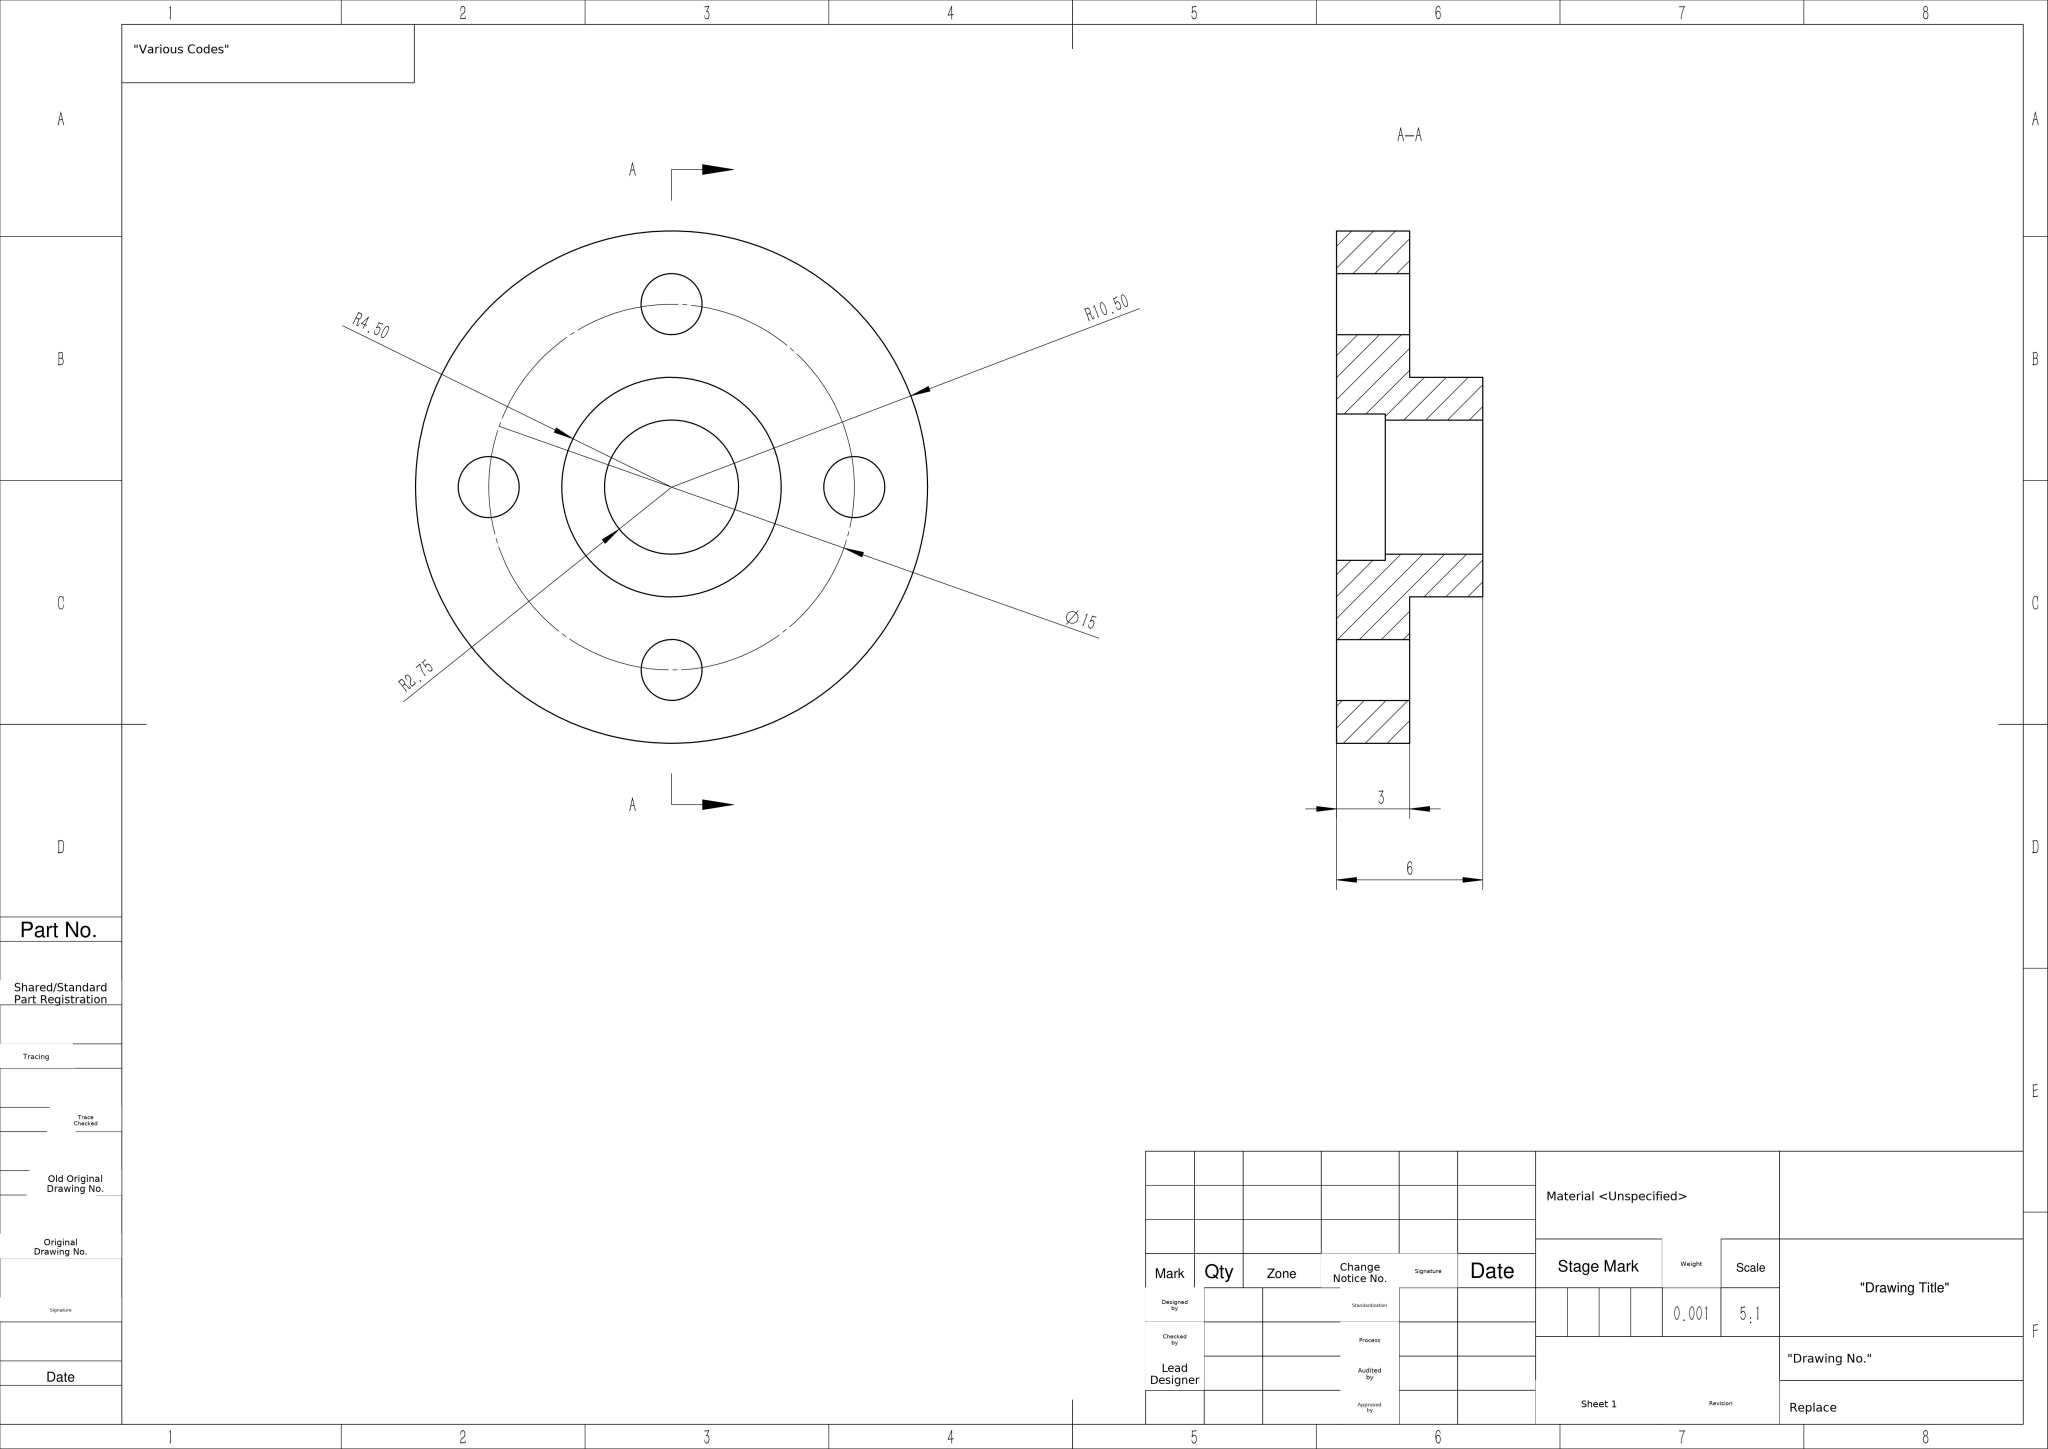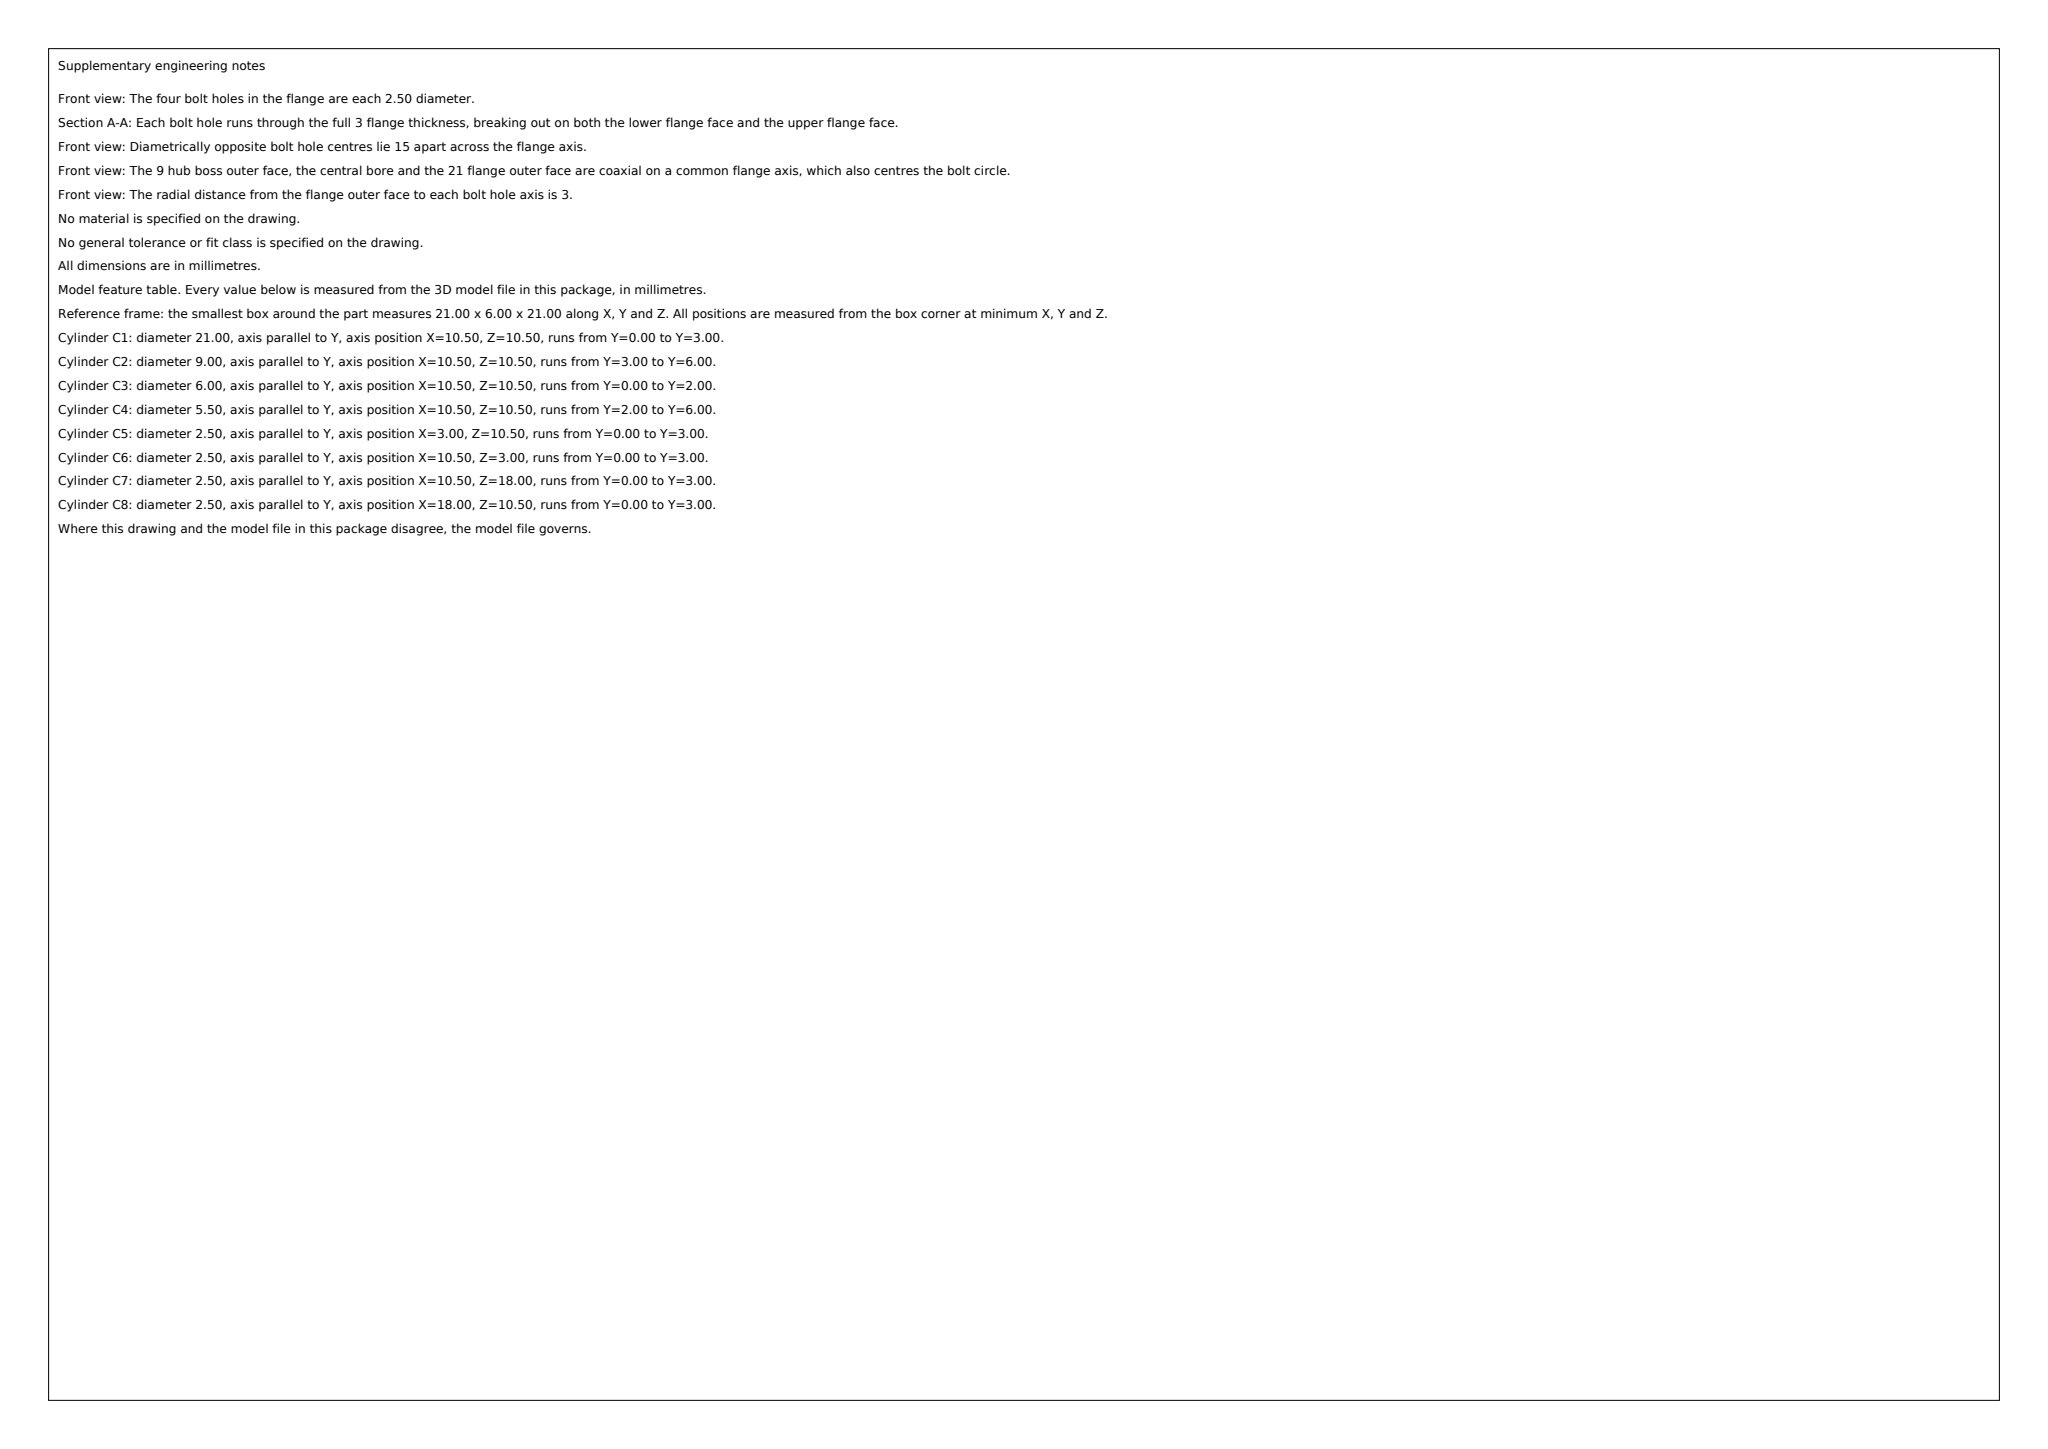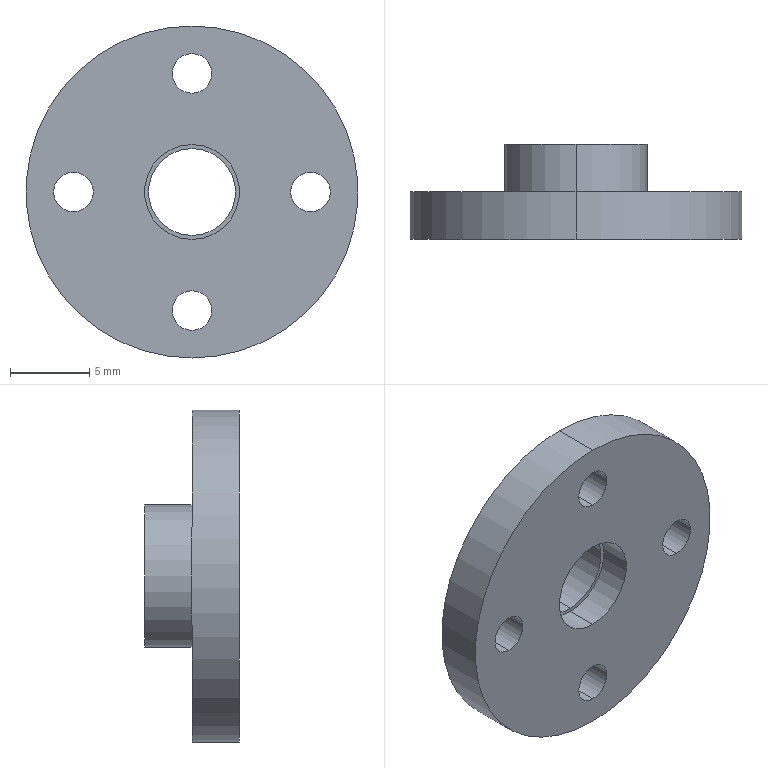Part | SolidWorks | mm | 1 solid | 20 faces | box 21 x 6 x 21 mm | volume 1019 mm3 | cylinder 16 | plane 4 | commonest cylinder face diameters 2.5 x8 6 x2 5.5 x2 9 x2 21 x2
Drawing notes:
Ø5.50 THRU; Ø6.00 DP 2 FROM FLANGE BACK FACE | from the solid: hole/bore dia 5.5 axis y from 2.0 to 6.0 at [10.5,10.5]; hole/bore dia 6.0 axis y from 0.0 to 2.0 at [10.5,10.5]
Ø5.50 THRU FROM Ø6.00 C'BORE FLOOR | from the solid: hole/bore dia 5.5, axis y at (10.5,10.5), from y=2.0 to 6.0 (thru hub end face at y=6); adjacent hole/bore dia 6.0 from y=0 to 2.0
STEP:
#1=CARTESIAN_POINT('',(-0.,3.,-6.25));
#2=VERTEX_POINT('',#1);
#3=CARTESIAN_POINT('',(-0.,0.,-6.25));
#4=VERTEX_POINT('',#3);
#5=CARTESIAN_POINT('',(-0.,6.,-6.25));
#6=DIRECTION('',(0.,-1.,0.));
#7=VECTOR('',#6,1000.);
#8=LINE('',#5,#7);
#9=EDGE_CURVE('',#2,#4,#8,.T.);
#10=ORIENTED_EDGE('',*,*,#9,.F.);
#11=CARTESIAN_POINT('',(-0.,3.,-8.75));
#12=VERTEX_POINT('',#11);
#13=CARTESIAN_POINT('',(-0.,3.,-7.5));
#14=DIRECTION('',(0.,1.,0.));
#15=DIRECTION('',(0.,0.,1.));
#16=AXIS2_PLACEMENT_3D('',#13,#14,#15);
#17=CIRCLE('',#16,1.25);
#18=EDGE_CURVE('',#2,#12,#17,.T.);
#19=ORIENTED_EDGE('',*,*,#18,.T.);
#20=CARTESIAN_POINT('',(-0.,0.,-8.75));
#21=VERTEX_POINT('',#20);
#22=CARTESIAN_POINT('',(-0.,6.,-8.75));
#23=DIRECTION('',(0.,-1.,0.));
#24=VECTOR('',#23,1000.);
#25=LINE('',#22,#24);
#26=EDGE_CURVE('',#12,#21,#25,.T.);
#27=ORIENTED_EDGE('',*,*,#26,.T.);
#28=CARTESIAN_POINT('',(-0.,0.,-7.5));
#29=DIRECTION('',(0.,-1.,0.));
#30=DIRECTION('',(-1.,0.,0.));
#31=AXIS2_PLACEMENT_3D('',#28,#29,#30);
#32=CIRCLE('',#31,1.25);
#33=EDGE_CURVE('',#21,#4,#32,.T.);
#34=ORIENTED_EDGE('',*,*,#33,.T.);
#35=EDGE_LOOP('',(#10,#19,#27,#34));
#36=FACE_OUTER_BOUND('',#35,.T.);
#37=CARTESIAN_POINT('',(-0.,6.,-7.5));
#38=DIRECTION('',(0.,-1.,0.));
#39=DIRECTION('',(0.,0.,-1.));
#40=AXIS2_PLACEMENT_3D('',#37,#38,#39);
#41=CYLINDRICAL_SURFACE('',#40,1.25);
#42=ADVANCED_FACE('',(#36),#41,.F.);
#43=CARTESIAN_POINT('',(-7.5,3.,1.25));
#44=VERTEX_POINT('',#43);
#45=CARTESIAN_POINT('',(-7.5,0.,1.25));
#46=VERTEX_POINT('',#45);
#47=CARTESIAN_POINT('',(-7.5,6.,1.25));
#48=DIRECTION('',(0.,-1.,0.));
#49=VECTOR('',#48,1000.);
#50=LINE('',#47,#49);
#51=EDGE_CURVE('',#44,#46,#50,.T.);
#52=ORIENTED_EDGE('',*,*,#51,.F.);
#53=CARTESIAN_POINT('',(-7.5,3.,-1.25));
#54=VERTEX_POINT('',#53);
#55=CARTESIAN_POINT('',(-7.5,3.,0.));
#56=DIRECTION('',(0.,1.,0.));
#57=DIRECTION('',(0.,0.,1.));
#58=AXIS2_PLACEMENT_3D('',#55,#56,#57);
#59=CIRCLE('',#58,1.25);
#60=EDGE_CURVE('',#44,#54,#59,.T.);
#61=ORIENTED_EDGE('',*,*,#60,.T.);
#62=CARTESIAN_POINT('',(-7.5,0.,-1.25));
#63=VERTEX_POINT('',#62);
#64=CARTESIAN_POINT('',(-7.5,6.,-1.25));
#65=DIRECTION('',(0.,-1.,0.));
#66=VECTOR('',#65,1000.);
#67=LINE('',#64,#66);
#68=EDGE_CURVE('',#54,#63,#67,.T.);
#69=ORIENTED_EDGE('',*,*,#68,.T.);
#70=CARTESIAN_POINT('',(-7.5,0.,0.));
#71=DIRECTION('',(0.,-1.,0.));
#72=DIRECTION('',(0.,0.,1.));
#73=AXIS2_PLACEMENT_3D('',#70,#71,#72);
#74=CIRCLE('',#73,1.25);
#75=EDGE_CURVE('',#63,#46,#74,.T.);
#76=ORIENTED_EDGE('',*,*,#75,.T.);
#77=EDGE_LOOP('',(#52,#61,#69,#76));
#78=FACE_OUTER_BOUND('',#77,.T.);
#79=CARTESIAN_POINT('',(-7.5,6.,0.));
#80=DIRECTION('',(0.,-1.,0.));
#81=DIRECTION('',(0.,0.,-1.));
#82=AXIS2_PLACEMENT_3D('',#79,#80,#81);
#83=CYLINDRICAL_SURFACE('',#82,1.25);
#84=ADVANCED_FACE('',(#78),#83,.F.);
#85=CARTESIAN_POINT('',(0.,3.,8.75));
#86=VERTEX_POINT('',#85);
#87=CARTESIAN_POINT('',(0.,0.,8.75));
#88=VERTEX_POINT('',#87);
#89=CARTESIAN_POINT('',(0.,6.,8.75));
#90=DIRECTION('',(0.,-1.,0.));
#91=VECTOR('',#90,1000.);
#92=LINE('',#89,#91);
#93=EDGE_CURVE('',#86,#88,#92,.T.);
#94=ORIENTED_EDGE('',*,*,#93,.F.);
#95=CARTESIAN_POINT('',(0.,3.,6.25));
#96=VERTEX_POINT('',#95);
#97=CARTESIAN_POINT('',(0.,3.,7.5));
#98=DIRECTION('',(0.,1.,0.));
#99=DIRECTION('',(0.,0.,1.));
#100=AXIS2_PLACEMENT_3D('',#97,#98,#99);
#101=CIRCLE('',#100,1.25);
#102=EDGE_CURVE('',#86,#96,#101,.T.);
#103=ORIENTED_EDGE('',*,*,#102,.T.);
#104=CARTESIAN_POINT('',(0.,0.,6.25));
#105=VERTEX_POINT('',#104);
#106=CARTESIAN_POINT('',(0.,6.,6.25));
#107=DIRECTION('',(0.,-1.,0.));
#108=VECTOR('',#107,1000.);
#109=LINE('',#106,#108);
#110=EDGE_CURVE('',#96,#105,#109,.T.);
#111=ORIENTED_EDGE('',*,*,#110,.T.);
#112=CARTESIAN_POINT('',(0.,0.,7.5));
#113=DIRECTION('',(0.,-1.,0.));
#114=DIRECTION('',(1.,0.,-0.));
#115=AXIS2_PLACEMENT_3D('',#112,#113,#114);
#116=CIRCLE('',#115,1.25);
#117=EDGE_CURVE('',#105,#88,#116,.T.);
#118=ORIENTED_EDGE('',*,*,#117,.T.);
#119=EDGE_LOOP('',(#94,#103,#111,#118));
#120=FACE_OUTER_BOUND('',#119,.T.);
#121=CARTESIAN_POINT('',(0.,6.,7.5));
#122=DIRECTION('',(0.,-1.,0.));
#123=DIRECTION('',(0.,0.,-1.));
#124=AXIS2_PLACEMENT_3D('',#121,#122,#123);
#125=CYLINDRICAL_SURFACE('',#124,1.25);
#126=ADVANCED_FACE('',(#120),#125,.F.);
#127=CARTESIAN_POINT('',(7.5,3.,1.25));
#128=VERTEX_POINT('',#127);
#129=CARTESIAN_POINT('',(7.5,0.,1.25));
#130=VERTEX_POINT('',#129);
#131=CARTESIAN_POINT('',(7.5,6.,1.25));
#132=DIRECTION('',(0.,-1.,0.));
#133=VECTOR('',#132,1000.);
#134=LINE('',#131,#133);
#135=EDGE_CURVE('',#128,#130,#134,.T.);
#136=ORIENTED_EDGE('',*,*,#135,.F.);
#137=CARTESIAN_POINT('',(7.5,3.,-1.25));
#138=VERTEX_POINT('',#137);
#139=CARTESIAN_POINT('',(7.5,3.,0.));
#140=DIRECTION('',(0.,1.,0.));
#141=DIRECTION('',(0.,0.,1.));
#142=AXIS2_PLACEMENT_3D('',#139,#140,#141);
#143=CIRCLE('',#142,1.25);
#144=EDGE_CURVE('',#128,#138,#143,.T.);
#145=ORIENTED_EDGE('',*,*,#144,.T.);
#146=CARTESIAN_POINT('',(7.5,0.,-1.25));
#147=VERTEX_POINT('',#146);
#148=CARTESIAN_POINT('',(7.5,6.,-1.25));
#149=DIRECTION('',(0.,-1.,0.));
#150=VECTOR('',#149,1000.);
#151=LINE('',#148,#150);
#152=EDGE_CURVE('',#138,#147,#151,.T.);
#153=ORIENTED_EDGE('',*,*,#152,.T.);
#154=CARTESIAN_POINT('',(7.5,0.,0.));
#155=DIRECTION('',(0.,-1.,0.));
#156=DIRECTION('',(0.,0.,-1.));
#157=AXIS2_PLACEMENT_3D('',#154,#155,#156);
#158=CIRCLE('',#157,1.25);
#159=EDGE_CURVE('',#147,#130,#158,.T.);
#160=ORIENTED_EDGE('',*,*,#159,.T.);
#161=EDGE_LOOP('',(#136,#145,#153,#160));
#162=FACE_OUTER_BOUND('',#161,.T.);
#163=CARTESIAN_POINT('',(7.5,6.,0.));
#164=DIRECTION('',(0.,-1.,0.));
#165=DIRECTION('',(0.,0.,-1.));
#166=AXIS2_PLACEMENT_3D('',#163,#164,#165);
#167=CYLINDRICAL_SURFACE('',#166,1.25);
#168=ADVANCED_FACE('',(#162),#167,.F.);
#169=CARTESIAN_POINT('',(0.,2.,3.));
#170=VERTEX_POINT('',#169);
#171=CARTESIAN_POINT('',(0.,0.,3.));
#172=VERTEX_POINT('',#171);
#173=CARTESIAN_POINT('',(0.,2.,3.));
#174=DIRECTION('',(0.,-1.,0.));
#175=VECTOR('',#174,1000.);
#176=LINE('',#173,#175);
#177=EDGE_CURVE('',#170,#172,#176,.T.);
#178=ORIENTED_EDGE('',*,*,#177,.F.);
#179=CARTESIAN_POINT('',(0.,2.,-3.));
#180=VERTEX_POINT('',#179);
#181=CARTESIAN_POINT('',(0.,2.,0.));
#182=DIRECTION('',(0.,-1.,0.));
#183=DIRECTION('',(0.,0.,-1.));
#184=AXIS2_PLACEMENT_3D('',#181,#182,#183);
#185=CIRCLE('',#184,3.);
#186=EDGE_CURVE('',#180,#170,#185,.T.);
#187=ORIENTED_EDGE('',*,*,#186,.F.);
#188=CARTESIAN_POINT('',(0.,0.,-3.));
#189=VERTEX_POINT('',#188);
#190=CARTESIAN_POINT('',(0.,2.,-3.));
#191=DIRECTION('',(0.,-1.,0.));
#192=VECTOR('',#191,1000.);
#193=LINE('',#190,#192);
#194=EDGE_CURVE('',#180,#189,#193,.T.);
#195=ORIENTED_EDGE('',*,*,#194,.T.);
#196=CARTESIAN_POINT('',(0.,0.,0.));
#197=DIRECTION('',(0.,-1.,0.));
#198=DIRECTION('',(0.,0.,-1.));
#199=AXIS2_PLACEMENT_3D('',#196,#197,#198);
#200=CIRCLE('',#199,3.);
#201=EDGE_CURVE('',#189,#172,#200,.T.);
#202=ORIENTED_EDGE('',*,*,#201,.T.);
#203=EDGE_LOOP('',(#178,#187,#195,#202));
#204=FACE_OUTER_BOUND('',#203,.T.);
#205=CARTESIAN_POINT('',(0.,2.,0.));
#206=DIRECTION('',(0.,-1.,0.));
#207=DIRECTION('',(0.,0.,-1.));
#208=AXIS2_PLACEMENT_3D('',#205,#206,#207);
#209=CYLINDRICAL_SURFACE('',#208,3.);
#210=ADVANCED_FACE('',(#204),#209,.F.);
#211=CARTESIAN_POINT('',(0.,2.,2.75));
#212=VERTEX_POINT('',#211);
#213=CARTESIAN_POINT('',(0.,2.,-2.75));
#214=VERTEX_POINT('',#213);
#215=CARTESIAN_POINT('',(0.,2.,0.));
#216=DIRECTION('',(0.,1.,0.));
#217=DIRECTION('',(0.,0.,1.));
#218=AXIS2_PLACEMENT_3D('',#215,#216,#217);
#219=CIRCLE('',#218,2.75);
#220=EDGE_CURVE('',#212,#214,#219,.T.);
#221=ORIENTED_EDGE('',*,*,#220,.T.);
#222=CARTESIAN_POINT('',(0.,2.,0.));
#223=DIRECTION('',(0.,1.,0.));
#224=DIRECTION('',(0.,0.,1.));
#225=AXIS2_PLACEMENT_3D('',#222,#223,#224);
#226=CIRCLE('',#225,2.75);
#227=EDGE_CURVE('',#214,#212,#226,.T.);
#228=ORIENTED_EDGE('',*,*,#227,.T.);
#229=EDGE_LOOP('',(#221,#228));
#230=FACE_BOUND('',#229,.T.);
#231=ORIENTED_EDGE('',*,*,#186,.T.);
#232=CARTESIAN_POINT('',(0.,2.,0.));
#233=DIRECTION('',(0.,-1.,0.));
#234=DIRECTION('',(0.,0.,-1.));
#235=AXIS2_PLACEMENT_3D('',#232,#233,#234);
#236=CIRCLE('',#235,3.);
#237=EDGE_CURVE('',#170,#180,#236,.T.);
#238=ORIENTED_EDGE('',*,*,#237,.T.);
#239=EDGE_LOOP('',(#231,#238));
#240=FACE_OUTER_BOUND('',#239,.T.);
#241=CARTESIAN_POINT('',(0.,2.,0.));
#242=DIRECTION('',(0.,-1.,0.));
#243=DIRECTION('',(0.,0.,-1.));
#244=AXIS2_PLACEMENT_3D('',#241,#242,#243);
#245=PLANE('',#244);
#246=ADVANCED_FACE('',(#230,#240),#245,.T.);
#247=CARTESIAN_POINT('',(0.,6.,-2.75));
#248=VERTEX_POINT('',#247);
#249=CARTESIAN_POINT('',(0.,2.,-2.75));
#250=DIRECTION('',(0.,1.,0.));
#251=VECTOR('',#250,1000.);
#252=LINE('',#249,#251);
#253=EDGE_CURVE('',#214,#248,#252,.T.);
#254=ORIENTED_EDGE('',*,*,#253,.F.);
#255=ORIENTED_EDGE('',*,*,#220,.F.);
#256=CARTESIAN_POINT('',(0.,6.,2.75));
#257=VERTEX_POINT('',#256);
#258=CARTESIAN_POINT('',(0.,2.,2.75));
#259=DIRECTION('',(0.,1.,0.));
#260=VECTOR('',#259,1000.);
#261=LINE('',#258,#260);
#262=EDGE_CURVE('',#212,#257,#261,.T.);
#263=ORIENTED_EDGE('',*,*,#262,.T.);
#264=CARTESIAN_POINT('',(0.,6.,0.));
#265=DIRECTION('',(0.,1.,0.));
#266=DIRECTION('',(0.,0.,1.));
#267=AXIS2_PLACEMENT_3D('',#264,#265,#266);
#268=CIRCLE('',#267,2.75);
#269=EDGE_CURVE('',#257,#248,#268,.T.);
#270=ORIENTED_EDGE('',*,*,#269,.T.);
#271=EDGE_LOOP('',(#254,#255,#263,#270));
#272=FACE_OUTER_BOUND('',#271,.T.);
#273=CARTESIAN_POINT('',(0.,2.,0.));
#274=DIRECTION('',(0.,1.,0.));
#275=DIRECTION('',(0.,0.,1.));
#276=AXIS2_PLACEMENT_3D('',#273,#274,#275);
#277=CYLINDRICAL_SURFACE('',#276,2.75);
#278=ADVANCED_FACE('',(#272),#277,.F.);
#279=ORIENTED_EDGE('',*,*,#269,.F.);
#280=CARTESIAN_POINT('',(0.,6.,0.));
#281=DIRECTION('',(0.,1.,0.));
#282=DIRECTION('',(0.,0.,1.));
#283=AXIS2_PLACEMENT_3D('',#280,#281,#282);
#284=CIRCLE('',#283,2.75);
#285=EDGE_CURVE('',#248,#257,#284,.T.);
#286=ORIENTED_EDGE('',*,*,#285,.F.);
#287=EDGE_LOOP('',(#279,#286));
#288=FACE_BOUND('',#287,.T.);
#289=CARTESIAN_POINT('',(0.,6.,-4.5));
#290=VERTEX_POINT('',#289);
#291=CARTESIAN_POINT('',(0.,6.,4.5));
#292=VERTEX_POINT('',#291);
#293=CARTESIAN_POINT('',(0.,6.,0.));
#294=DIRECTION('',(0.,1.,0.));
#295=DIRECTION('',(0.,0.,1.));
#296=AXIS2_PLACEMENT_3D('',#293,#294,#295);
#297=CIRCLE('',#296,4.5);
#298=EDGE_CURVE('',#290,#292,#297,.T.);
#299=ORIENTED_EDGE('',*,*,#298,.T.);
#300=CARTESIAN_POINT('',(0.,6.,0.));
#301=DIRECTION('',(0.,1.,0.));
#302=DIRECTION('',(0.,0.,1.));
#303=AXIS2_PLACEMENT_3D('',#300,#301,#302);
#304=CIRCLE('',#303,4.5);
#305=EDGE_CURVE('',#292,#290,#304,.T.);
#306=ORIENTED_EDGE('',*,*,#305,.T.);
#307=EDGE_LOOP('',(#299,#306));
#308=FACE_OUTER_BOUND('',#307,.T.);
#309=CARTESIAN_POINT('',(0.,6.,0.));
#310=DIRECTION('',(0.,1.,0.));
#311=DIRECTION('',(1.,0.,0.));
#312=AXIS2_PLACEMENT_3D('',#309,#310,#311);
#313=PLANE('',#312);
#314=ADVANCED_FACE('',(#288,#308),#313,.T.);
#315=CARTESIAN_POINT('',(0.,3.,4.5));
#316=VERTEX_POINT('',#315);
#317=CARTESIAN_POINT('',(0.,6.,4.5));
#318=DIRECTION('',(0.,-1.,0.));
#319=VECTOR('',#318,1000.);
#320=LINE('',#317,#319);
#321=EDGE_CURVE('',#292,#316,#320,.T.);
#322=ORIENTED_EDGE('',*,*,#321,.F.);
#323=ORIENTED_EDGE('',*,*,#298,.F.);
#324=CARTESIAN_POINT('',(0.,3.,-4.5));
#325=VERTEX_POINT('',#324);
#326=CARTESIAN_POINT('',(0.,6.,-4.5));
#327=DIRECTION('',(0.,-1.,0.));
#328=VECTOR('',#327,1000.);
#329=LINE('',#326,#328);
#330=EDGE_CURVE('',#290,#325,#329,.T.);
#331=ORIENTED_EDGE('',*,*,#330,.T.);
#332=CARTESIAN_POINT('',(0.,3.,0.));
#333=DIRECTION('',(0.,1.,0.));
#334=DIRECTION('',(0.,0.,1.));
#335=AXIS2_PLACEMENT_3D('',#332,#333,#334);
#336=CIRCLE('',#335,4.5);
#337=EDGE_CURVE('',#325,#316,#336,.T.);
#338=ORIENTED_EDGE('',*,*,#337,.T.);
#339=EDGE_LOOP('',(#322,#323,#331,#338));
#340=FACE_OUTER_BOUND('',#339,.T.);
#341=CARTESIAN_POINT('',(0.,6.,0.));
#342=DIRECTION('',(0.,-1.,0.));
#343=DIRECTION('',(0.,0.,-1.));
#344=AXIS2_PLACEMENT_3D('',#341,#342,#343);
#345=CYLINDRICAL_SURFACE('',#344,4.5);
#346=ADVANCED_FACE('',(#340),#345,.T.);
#347=ORIENTED_EDGE('',*,*,#201,.F.);
#348=CARTESIAN_POINT('',(0.,0.,0.));
#349=DIRECTION('',(0.,-1.,0.));
#350=DIRECTION('',(0.,0.,-1.));
#351=AXIS2_PLACEMENT_3D('',#348,#349,#350);
#352=CIRCLE('',#351,3.);
#353=EDGE_CURVE('',#172,#189,#352,.T.);
#354=ORIENTED_EDGE('',*,*,#353,.F.);
#355=EDGE_LOOP('',(#347,#354));
#356=FACE_BOUND('',#355,.T.);
#357=ORIENTED_EDGE('',*,*,#159,.F.);
#358=CARTESIAN_POINT('',(7.5,0.,0.));
#359=DIRECTION('',(0.,-1.,0.));
#360=DIRECTION('',(0.,0.,-1.));
#361=AXIS2_PLACEMENT_3D('',#358,#359,#360);
#362=CIRCLE('',#361,1.25);
#363=EDGE_CURVE('',#130,#147,#362,.T.);
#364=ORIENTED_EDGE('',*,*,#363,.F.);
#365=EDGE_LOOP('',(#357,#364));
#366=FACE_BOUND('',#365,.T.);
#367=ORIENTED_EDGE('',*,*,#117,.F.);
#368=CARTESIAN_POINT('',(0.,0.,7.5));
#369=DIRECTION('',(0.,-1.,0.));
#370=DIRECTION('',(1.,0.,-0.));
#371=AXIS2_PLACEMENT_3D('',#368,#369,#370);
#372=CIRCLE('',#371,1.25);
#373=EDGE_CURVE('',#88,#105,#372,.T.);
#374=ORIENTED_EDGE('',*,*,#373,.F.);
#375=EDGE_LOOP('',(#367,#374));
#376=FACE_BOUND('',#375,.T.);
#377=ORIENTED_EDGE('',*,*,#75,.F.);
#378=CARTESIAN_POINT('',(-7.5,0.,0.));
#379=DIRECTION('',(0.,-1.,0.));
#380=DIRECTION('',(0.,0.,1.));
#381=AXIS2_PLACEMENT_3D('',#378,#379,#380);
#382=CIRCLE('',#381,1.25);
#383=EDGE_CURVE('',#46,#63,#382,.T.);
#384=ORIENTED_EDGE('',*,*,#383,.F.);
#385=EDGE_LOOP('',(#377,#384));
#386=FACE_BOUND('',#385,.T.);
#387=ORIENTED_EDGE('',*,*,#33,.F.);
#388=CARTESIAN_POINT('',(-0.,0.,-7.5));
#389=DIRECTION('',(0.,-1.,0.));
#390=DIRECTION('',(-1.,0.,0.));
#391=AXIS2_PLACEMENT_3D('',#388,#389,#390);
#392=CIRCLE('',#391,1.25);
#393=EDGE_CURVE('',#4,#21,#392,.T.);
#394=ORIENTED_EDGE('',*,*,#393,.F.);
#395=EDGE_LOOP('',(#387,#394));
#396=FACE_BOUND('',#395,.T.);
#397=CARTESIAN_POINT('',(0.,0.,-10.5));
#398=VERTEX_POINT('',#397);
#399=CARTESIAN_POINT('',(0.,0.,10.5));
#400=VERTEX_POINT('',#399);
#401=CARTESIAN_POINT('',(0.,0.,0.));
#402=DIRECTION('',(0.,1.,0.));
#403=DIRECTION('',(0.,0.,1.));
#404=AXIS2_PLACEMENT_3D('',#401,#402,#403);
#405=CIRCLE('',#404,10.5);
#406=EDGE_CURVE('',#398,#400,#405,.T.);
#407=ORIENTED_EDGE('',*,*,#406,.F.);
#408=CARTESIAN_POINT('',(0.,0.,0.));
#409=DIRECTION('',(0.,1.,0.));
#410=DIRECTION('',(0.,0.,1.));
#411=AXIS2_PLACEMENT_3D('',#408,#409,#410);
#412=CIRCLE('',#411,10.5);
#413=EDGE_CURVE('',#400,#398,#412,.T.);
#414=ORIENTED_EDGE('',*,*,#413,.F.);
#415=EDGE_LOOP('',(#407,#414));
#416=FACE_OUTER_BOUND('',#415,.T.);
#417=CARTESIAN_POINT('',(0.,0.,0.));
#418=DIRECTION('',(0.,1.,0.));
#419=DIRECTION('',(1.,0.,0.));
#420=AXIS2_PLACEMENT_3D('',#417,#418,#419);
#421=PLANE('',#420);
#422=ADVANCED_FACE('',(#356,#366,#376,#386,#396,#416),#421,.F.);
#423=ORIENTED_EDGE('',*,*,#337,.F.);
#424=CARTESIAN_POINT('',(0.,3.,0.));
#425=DIRECTION('',(0.,1.,0.));
#426=DIRECTION('',(0.,0.,1.));
#427=AXIS2_PLACEMENT_3D('',#424,#425,#426);
#428=CIRCLE('',#427,4.5);
#429=EDGE_CURVE('',#316,#325,#428,.T.);
#430=ORIENTED_EDGE('',*,*,#429,.F.);
#431=EDGE_LOOP('',(#423,#430));
#432=FACE_BOUND('',#431,.T.);
#433=CARTESIAN_POINT('',(7.5,3.,0.));
#434=DIRECTION('',(0.,1.,0.));
#435=DIRECTION('',(0.,0.,1.));
#436=AXIS2_PLACEMENT_3D('',#433,#434,#435);
#437=CIRCLE('',#436,1.25);
#438=EDGE_CURVE('',#138,#128,#437,.T.);
#439=ORIENTED_EDGE('',*,*,#438,.F.);
#440=ORIENTED_EDGE('',*,*,#144,.F.);
#441=EDGE_LOOP('',(#439,#440));
#442=FACE_BOUND('',#441,.T.);
#443=CARTESIAN_POINT('',(0.,3.,7.5));
#444=DIRECTION('',(0.,1.,0.));
#445=DIRECTION('',(0.,0.,1.));
#446=AXIS2_PLACEMENT_3D('',#443,#444,#445);
#447=CIRCLE('',#446,1.25);
#448=EDGE_CURVE('',#96,#86,#447,.T.);
#449=ORIENTED_EDGE('',*,*,#448,.F.);
#450=ORIENTED_EDGE('',*,*,#102,.F.);
#451=EDGE_LOOP('',(#449,#450));
#452=FACE_BOUND('',#451,.T.);
#453=CARTESIAN_POINT('',(-7.5,3.,0.));
#454=DIRECTION('',(0.,1.,0.));
#455=DIRECTION('',(0.,0.,1.));
#456=AXIS2_PLACEMENT_3D('',#453,#454,#455);
#457=CIRCLE('',#456,1.25);
#458=EDGE_CURVE('',#54,#44,#457,.T.);
#459=ORIENTED_EDGE('',*,*,#458,.F.);
#460=ORIENTED_EDGE('',*,*,#60,.F.);
#461=EDGE_LOOP('',(#459,#460));
#462=FACE_BOUND('',#461,.T.);
#463=CARTESIAN_POINT('',(-0.,3.,-7.5));
#464=DIRECTION('',(0.,1.,0.));
#465=DIRECTION('',(0.,0.,1.));
#466=AXIS2_PLACEMENT_3D('',#463,#464,#465);
#467=CIRCLE('',#466,1.25);
#468=EDGE_CURVE('',#12,#2,#467,.T.);
#469=ORIENTED_EDGE('',*,*,#468,.F.);
#470=ORIENTED_EDGE('',*,*,#18,.F.);
#471=EDGE_LOOP('',(#469,#470));
#472=FACE_BOUND('',#471,.T.);
#473=CARTESIAN_POINT('',(0.,3.,-10.5));
#474=VERTEX_POINT('',#473);
#475=CARTESIAN_POINT('',(0.,3.,10.5));
#476=VERTEX_POINT('',#475);
#477=CARTESIAN_POINT('',(0.,3.,0.));
#478=DIRECTION('',(0.,1.,0.));
#479=DIRECTION('',(0.,0.,1.));
#480=AXIS2_PLACEMENT_3D('',#477,#478,#479);
#481=CIRCLE('',#480,10.5);
#482=EDGE_CURVE('',#474,#476,#481,.T.);
#483=ORIENTED_EDGE('',*,*,#482,.T.);
#484=CARTESIAN_POINT('',(0.,3.,0.));
#485=DIRECTION('',(0.,1.,0.));
#486=DIRECTION('',(0.,0.,1.));
#487=AXIS2_PLACEMENT_3D('',#484,#485,#486);
#488=CIRCLE('',#487,10.5);
#489=EDGE_CURVE('',#476,#474,#488,.T.);
#490=ORIENTED_EDGE('',*,*,#489,.T.);
#491=EDGE_LOOP('',(#483,#490));
#492=FACE_OUTER_BOUND('',#491,.T.);
#493=CARTESIAN_POINT('',(0.,3.,0.));
#494=DIRECTION('',(0.,1.,0.));
#495=DIRECTION('',(1.,0.,0.));
#496=AXIS2_PLACEMENT_3D('',#493,#494,#495);
#497=PLANE('',#496);
#498=ADVANCED_FACE('',(#432,#442,#452,#462,#472,#492),#497,.T.);
#499=CARTESIAN_POINT('',(0.,3.,10.5));
#500=DIRECTION('',(0.,-1.,0.));
#501=VECTOR('',#500,1000.);
#502=LINE('',#499,#501);
#503=EDGE_CURVE('',#476,#400,#502,.T.);
#504=ORIENTED_EDGE('',*,*,#503,.F.);
#505=ORIENTED_EDGE('',*,*,#482,.F.);
#506=CARTESIAN_POINT('',(0.,3.,-10.5));
#507=DIRECTION('',(0.,-1.,0.));
#508=VECTOR('',#507,1000.);
#509=LINE('',#506,#508);
#510=EDGE_CURVE('',#474,#398,#509,.T.);
#511=ORIENTED_EDGE('',*,*,#510,.T.);
#512=ORIENTED_EDGE('',*,*,#406,.T.);
#513=EDGE_LOOP('',(#504,#505,#511,#512));
#514=FACE_OUTER_BOUND('',#513,.T.);
#515=CARTESIAN_POINT('',(0.,3.,0.));
#516=DIRECTION('',(0.,-1.,0.));
#517=DIRECTION('',(0.,0.,-1.));
#518=AXIS2_PLACEMENT_3D('',#515,#516,#517);
#519=CYLINDRICAL_SURFACE('',#518,10.5);
#520=ADVANCED_FACE('',(#514),#519,.T.);
#521=ORIENTED_EDGE('',*,*,#489,.F.);
#522=ORIENTED_EDGE('',*,*,#503,.T.);
#523=ORIENTED_EDGE('',*,*,#413,.T.);
#524=ORIENTED_EDGE('',*,*,#510,.F.);
#525=EDGE_LOOP('',(#521,#522,#523,#524));
#526=FACE_OUTER_BOUND('',#525,.T.);
#527=CARTESIAN_POINT('',(0.,3.,0.));
#528=DIRECTION('',(0.,-1.,0.));
#529=DIRECTION('',(0.,0.,-1.));
#530=AXIS2_PLACEMENT_3D('',#527,#528,#529);
#531=CYLINDRICAL_SURFACE('',#530,10.5);
#532=ADVANCED_FACE('',(#526),#531,.T.);
#533=ORIENTED_EDGE('',*,*,#305,.F.);
#534=ORIENTED_EDGE('',*,*,#321,.T.);
#535=ORIENTED_EDGE('',*,*,#429,.T.);
#536=ORIENTED_EDGE('',*,*,#330,.F.);
#537=EDGE_LOOP('',(#533,#534,#535,#536));
#538=FACE_OUTER_BOUND('',#537,.T.);
#539=CARTESIAN_POINT('',(0.,6.,0.));
#540=DIRECTION('',(0.,-1.,0.));
#541=DIRECTION('',(0.,0.,-1.));
#542=AXIS2_PLACEMENT_3D('',#539,#540,#541);
#543=CYLINDRICAL_SURFACE('',#542,4.5);
#544=ADVANCED_FACE('',(#538),#543,.T.);
#545=ORIENTED_EDGE('',*,*,#227,.F.);
#546=ORIENTED_EDGE('',*,*,#253,.T.);
#547=ORIENTED_EDGE('',*,*,#285,.T.);
#548=ORIENTED_EDGE('',*,*,#262,.F.);
#549=EDGE_LOOP('',(#545,#546,#547,#548));
#550=FACE_OUTER_BOUND('',#549,.T.);
#551=CARTESIAN_POINT('',(0.,2.,0.));
#552=DIRECTION('',(0.,1.,0.));
#553=DIRECTION('',(0.,0.,1.));
#554=AXIS2_PLACEMENT_3D('',#551,#552,#553);
#555=CYLINDRICAL_SURFACE('',#554,2.75);
#556=ADVANCED_FACE('',(#550),#555,.F.);
#557=ORIENTED_EDGE('',*,*,#237,.F.);
#558=ORIENTED_EDGE('',*,*,#177,.T.);
#559=ORIENTED_EDGE('',*,*,#353,.T.);
#560=ORIENTED_EDGE('',*,*,#194,.F.);
#561=EDGE_LOOP('',(#557,#558,#559,#560));
#562=FACE_OUTER_BOUND('',#561,.T.);
#563=CARTESIAN_POINT('',(0.,2.,0.));
#564=DIRECTION('',(0.,-1.,0.));
#565=DIRECTION('',(0.,0.,-1.));
#566=AXIS2_PLACEMENT_3D('',#563,#564,#565);
#567=CYLINDRICAL_SURFACE('',#566,3.);
#568=ADVANCED_FACE('',(#562),#567,.F.);
#569=ORIENTED_EDGE('',*,*,#438,.T.);
#570=ORIENTED_EDGE('',*,*,#135,.T.);
#571=ORIENTED_EDGE('',*,*,#363,.T.);
#572=ORIENTED_EDGE('',*,*,#152,.F.);
#573=EDGE_LOOP('',(#569,#570,#571,#572));
#574=FACE_OUTER_BOUND('',#573,.T.);
#575=CARTESIAN_POINT('',(7.5,6.,0.));
#576=DIRECTION('',(0.,-1.,0.));
#577=DIRECTION('',(0.,0.,-1.));
#578=AXIS2_PLACEMENT_3D('',#575,#576,#577);
#579=CYLINDRICAL_SURFACE('',#578,1.25);
#580=ADVANCED_FACE('',(#574),#579,.F.);
#581=ORIENTED_EDGE('',*,*,#448,.T.);
#582=ORIENTED_EDGE('',*,*,#93,.T.);
#583=ORIENTED_EDGE('',*,*,#373,.T.);
#584=ORIENTED_EDGE('',*,*,#110,.F.);
#585=EDGE_LOOP('',(#581,#582,#583,#584));
#586=FACE_OUTER_BOUND('',#585,.T.);
#587=CARTESIAN_POINT('',(0.,6.,7.5));
#588=DIRECTION('',(0.,-1.,0.));
#589=DIRECTION('',(0.,0.,-1.));
#590=AXIS2_PLACEMENT_3D('',#587,#588,#589);
#591=CYLINDRICAL_SURFACE('',#590,1.25);
#592=ADVANCED_FACE('',(#586),#591,.F.);
#593=ORIENTED_EDGE('',*,*,#458,.T.);
#594=ORIENTED_EDGE('',*,*,#51,.T.);
#595=ORIENTED_EDGE('',*,*,#383,.T.);
#596=ORIENTED_EDGE('',*,*,#68,.F.);
#597=EDGE_LOOP('',(#593,#594,#595,#596));
#598=FACE_OUTER_BOUND('',#597,.T.);
#599=CARTESIAN_POINT('',(-7.5,6.,0.));
#600=DIRECTION('',(0.,-1.,0.));
#601=DIRECTION('',(0.,0.,-1.));
#602=AXIS2_PLACEMENT_3D('',#599,#600,#601);
#603=CYLINDRICAL_SURFACE('',#602,1.25);
#604=ADVANCED_FACE('',(#598),#603,.F.);
#605=ORIENTED_EDGE('',*,*,#468,.T.);
#606=ORIENTED_EDGE('',*,*,#9,.T.);
#607=ORIENTED_EDGE('',*,*,#393,.T.);
#608=ORIENTED_EDGE('',*,*,#26,.F.);
#609=EDGE_LOOP('',(#605,#606,#607,#608));
#610=FACE_OUTER_BOUND('',#609,.T.);
#611=CARTESIAN_POINT('',(-0.,6.,-7.5));
#612=DIRECTION('',(0.,-1.,0.));
#613=DIRECTION('',(0.,0.,-1.));
#614=AXIS2_PLACEMENT_3D('',#611,#612,#613);
#615=CYLINDRICAL_SURFACE('',#614,1.25);
#616=ADVANCED_FACE('',(#610),#615,.F.);
#617=CLOSED_SHELL('',(#42,#84,#126,#168,#210,#246,#278,#314,#346,#422,#498,#520,#532,#544,#556,#568,#580,#592,#604,#616));
#618=MANIFOLD_SOLID_BREP('',#617);
#619=CARTESIAN_POINT('',(0.,0.,0.));
#620=DIRECTION('',(0.,0.,1.));
#621=DIRECTION('',(1.,0.,0.));
#622=AXIS2_PLACEMENT_3D('',#619,#620,#621);
#623=(LENGTH_UNIT()NAMED_UNIT(*)SI_UNIT(.MILLI.,.METRE.));
#624=UNCERTAINTY_MEASURE_WITH_UNIT(LENGTH_MEASURE(0.00001),#623,'','');
#625=(NAMED_UNIT(*)PLANE_ANGLE_UNIT()SI_UNIT($,.RADIAN.));
#626=(NAMED_UNIT(*)SI_UNIT($,.STERADIAN.)SOLID_ANGLE_UNIT());
#627=(GEOMETRIC_REPRESENTATION_CONTEXT(3)GLOBAL_UNCERTAINTY_ASSIGNED_CONTEXT((#624))GLOBAL_UNIT_ASSIGNED_CONTEXT((#623,#625,#626))REPRESENTATION_CONTEXT('',''));
#628=ADVANCED_BREP_SHAPE_REPRESENTATION('',(#618,#622),#627);